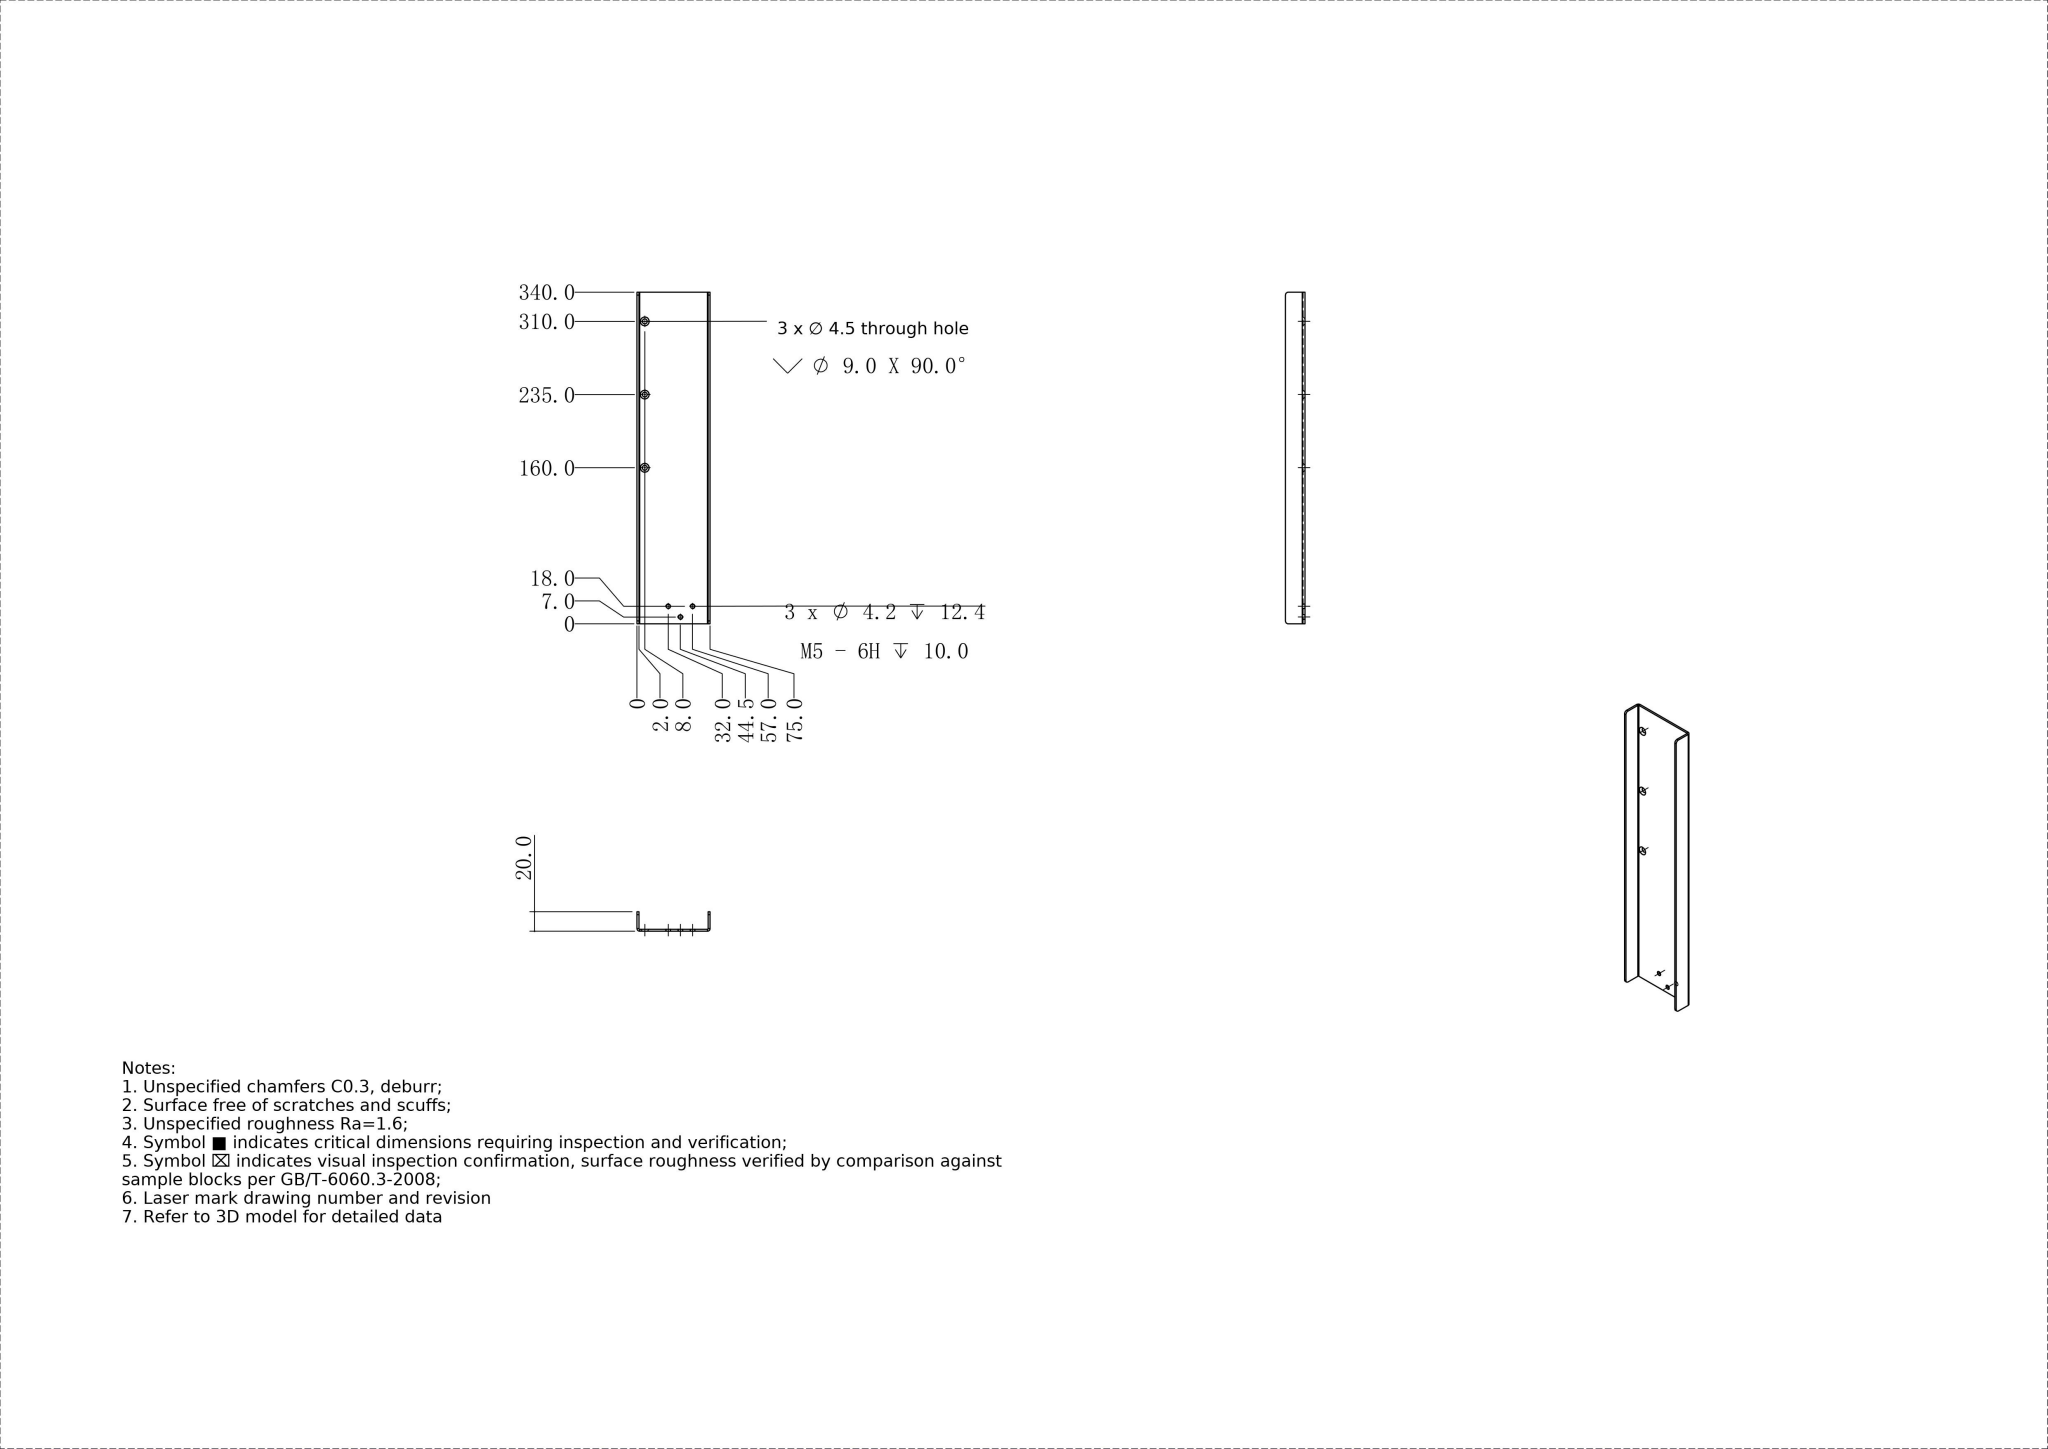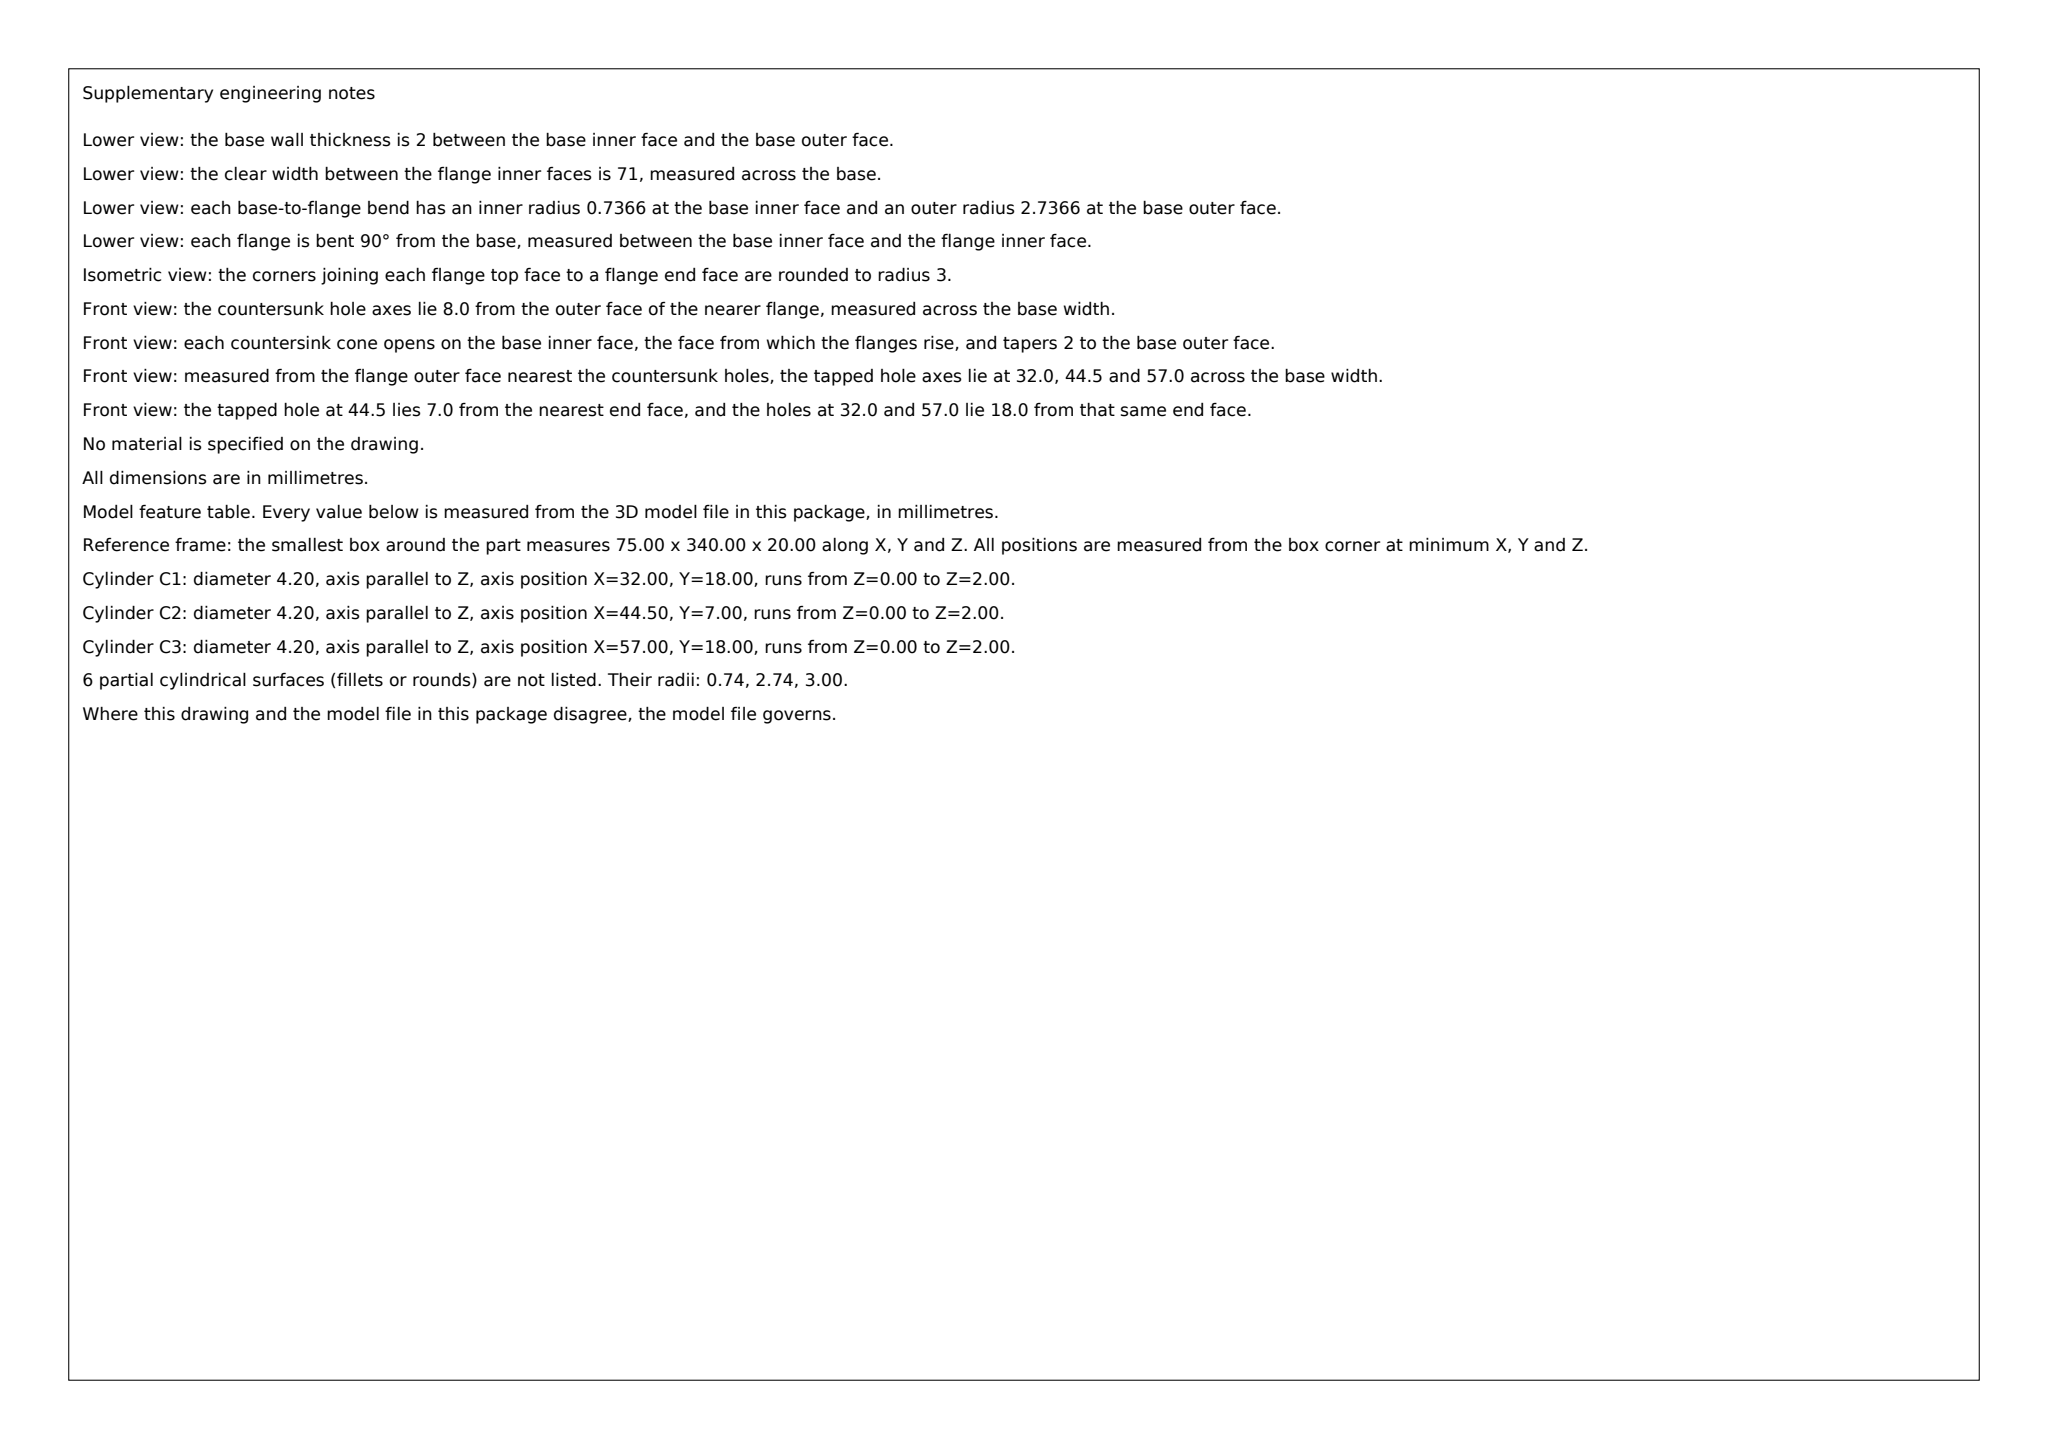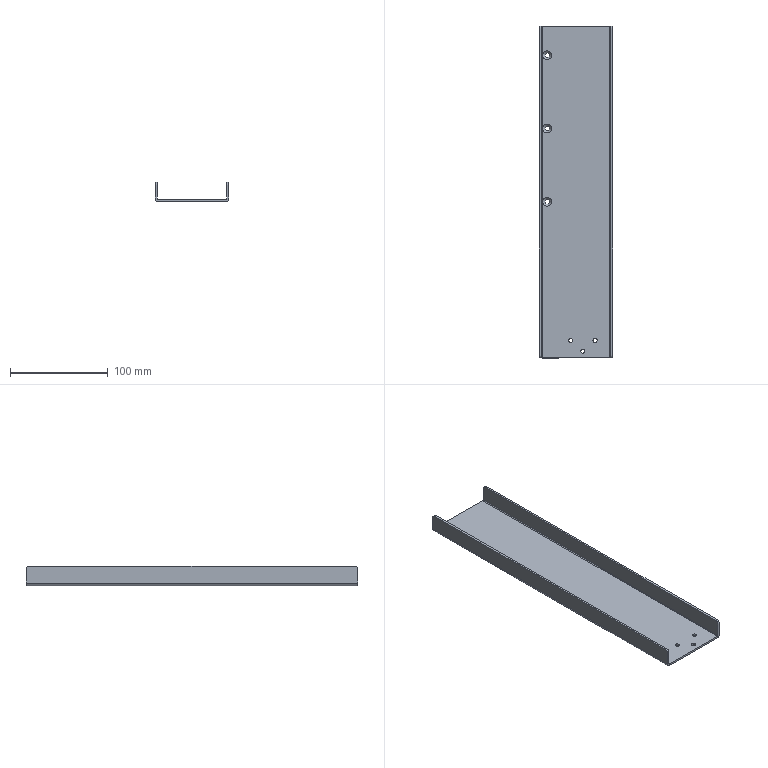Part | SolidWorks | mm | 1 solid | 38 faces | box 75 x 340 x 20 mm | volume 74133 mm3 | plane 18 | cylinder 14 | cone 6 | commonest cylinder face diameters 4.2 x6 6 x4 5.473 x2 1.473 x2